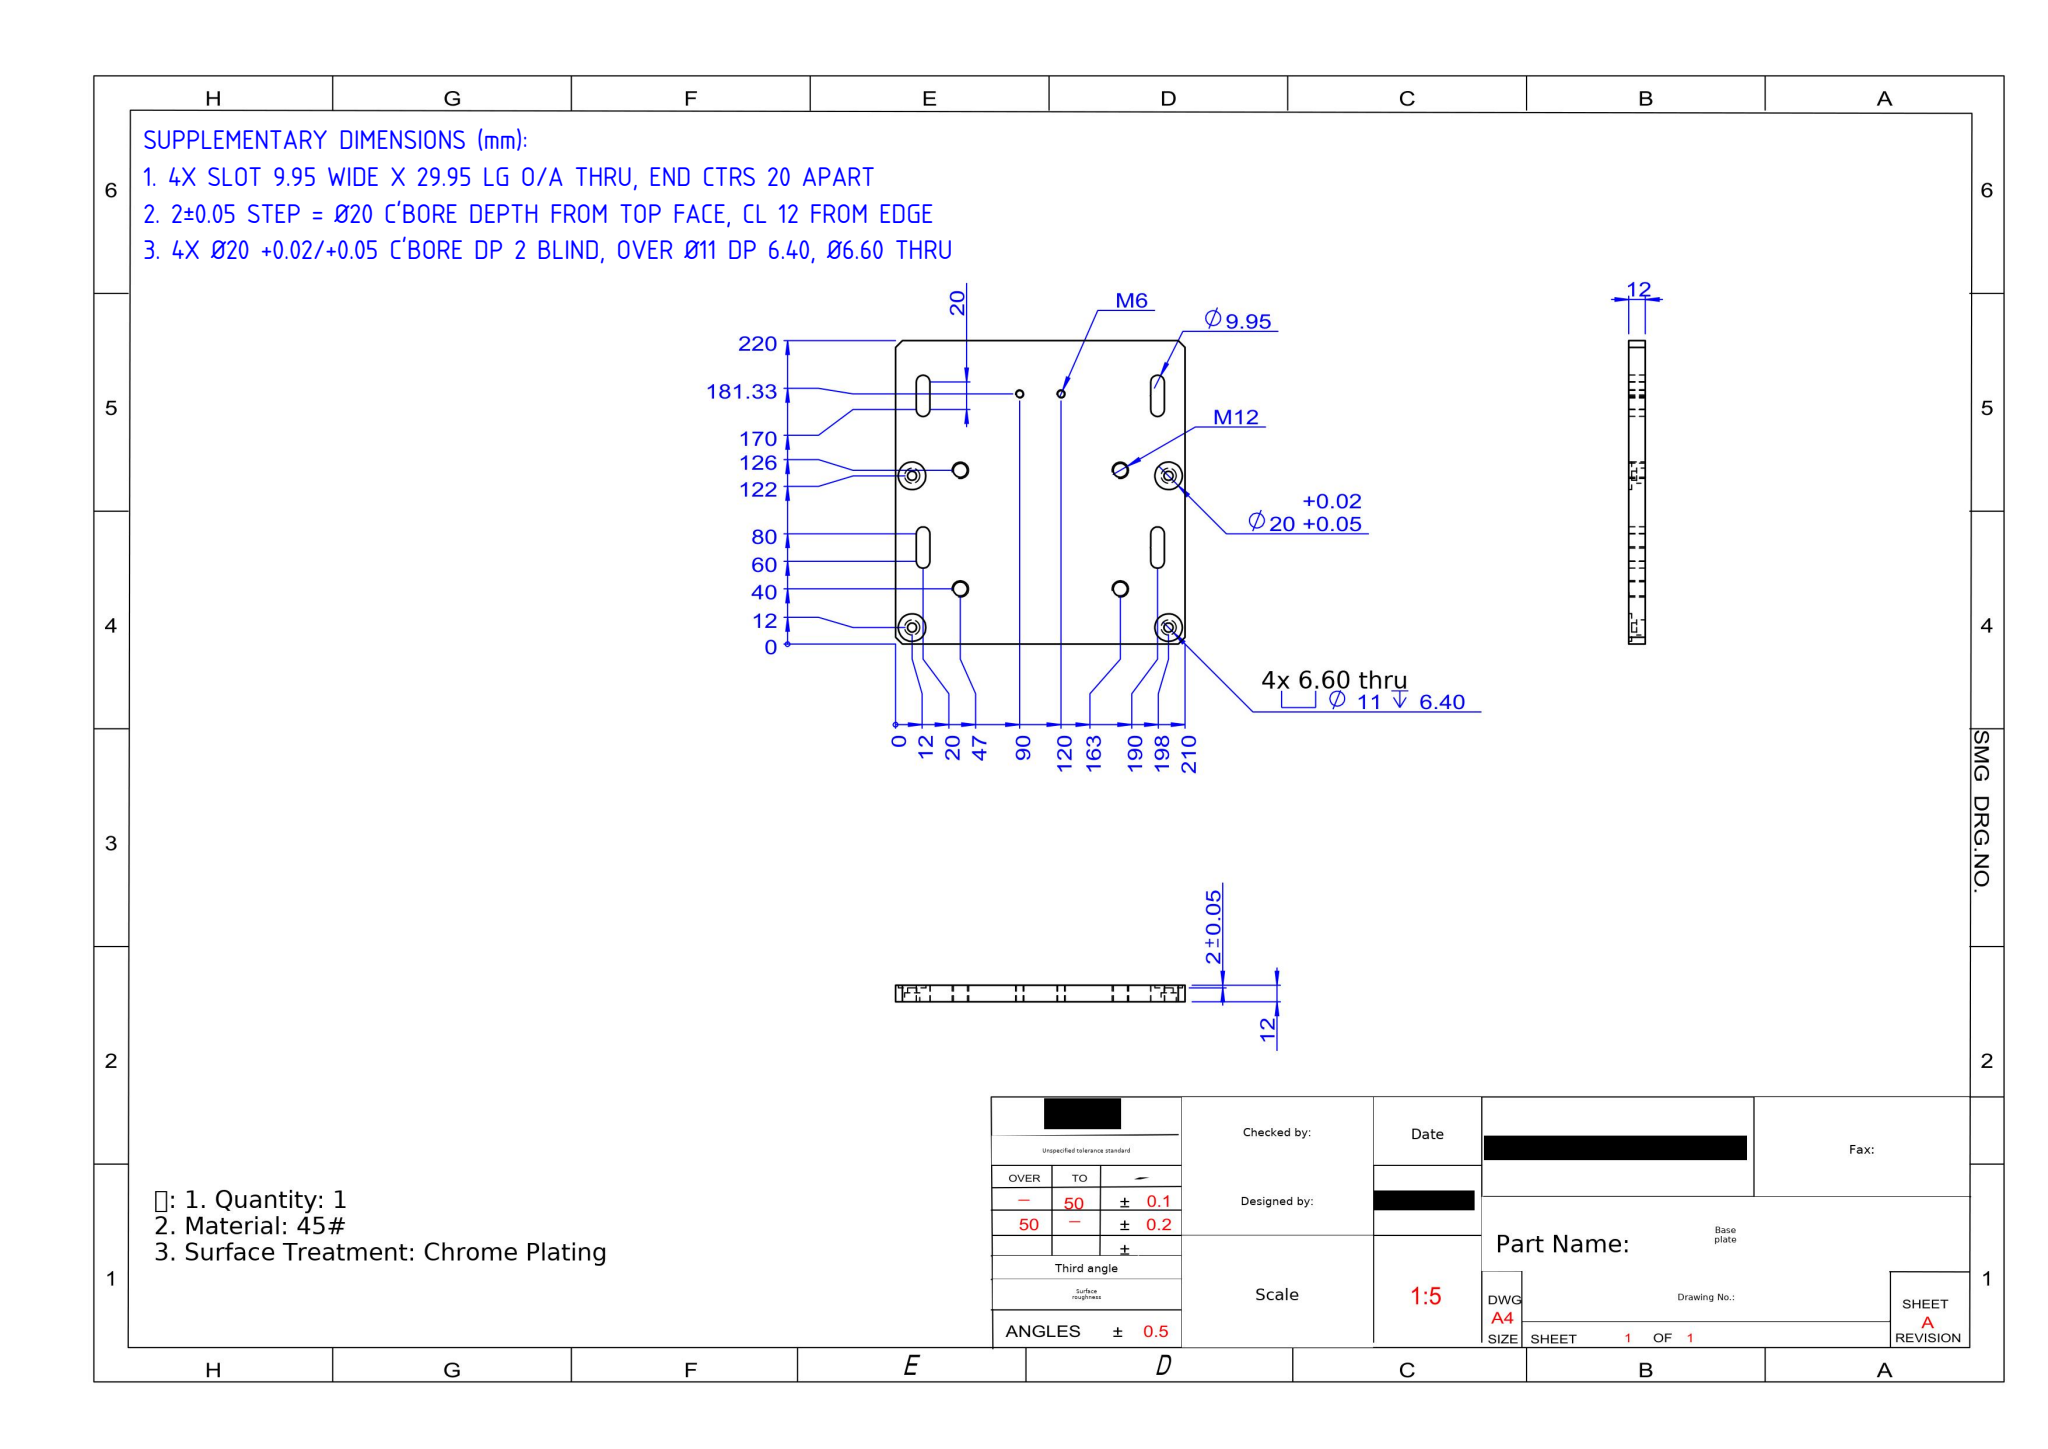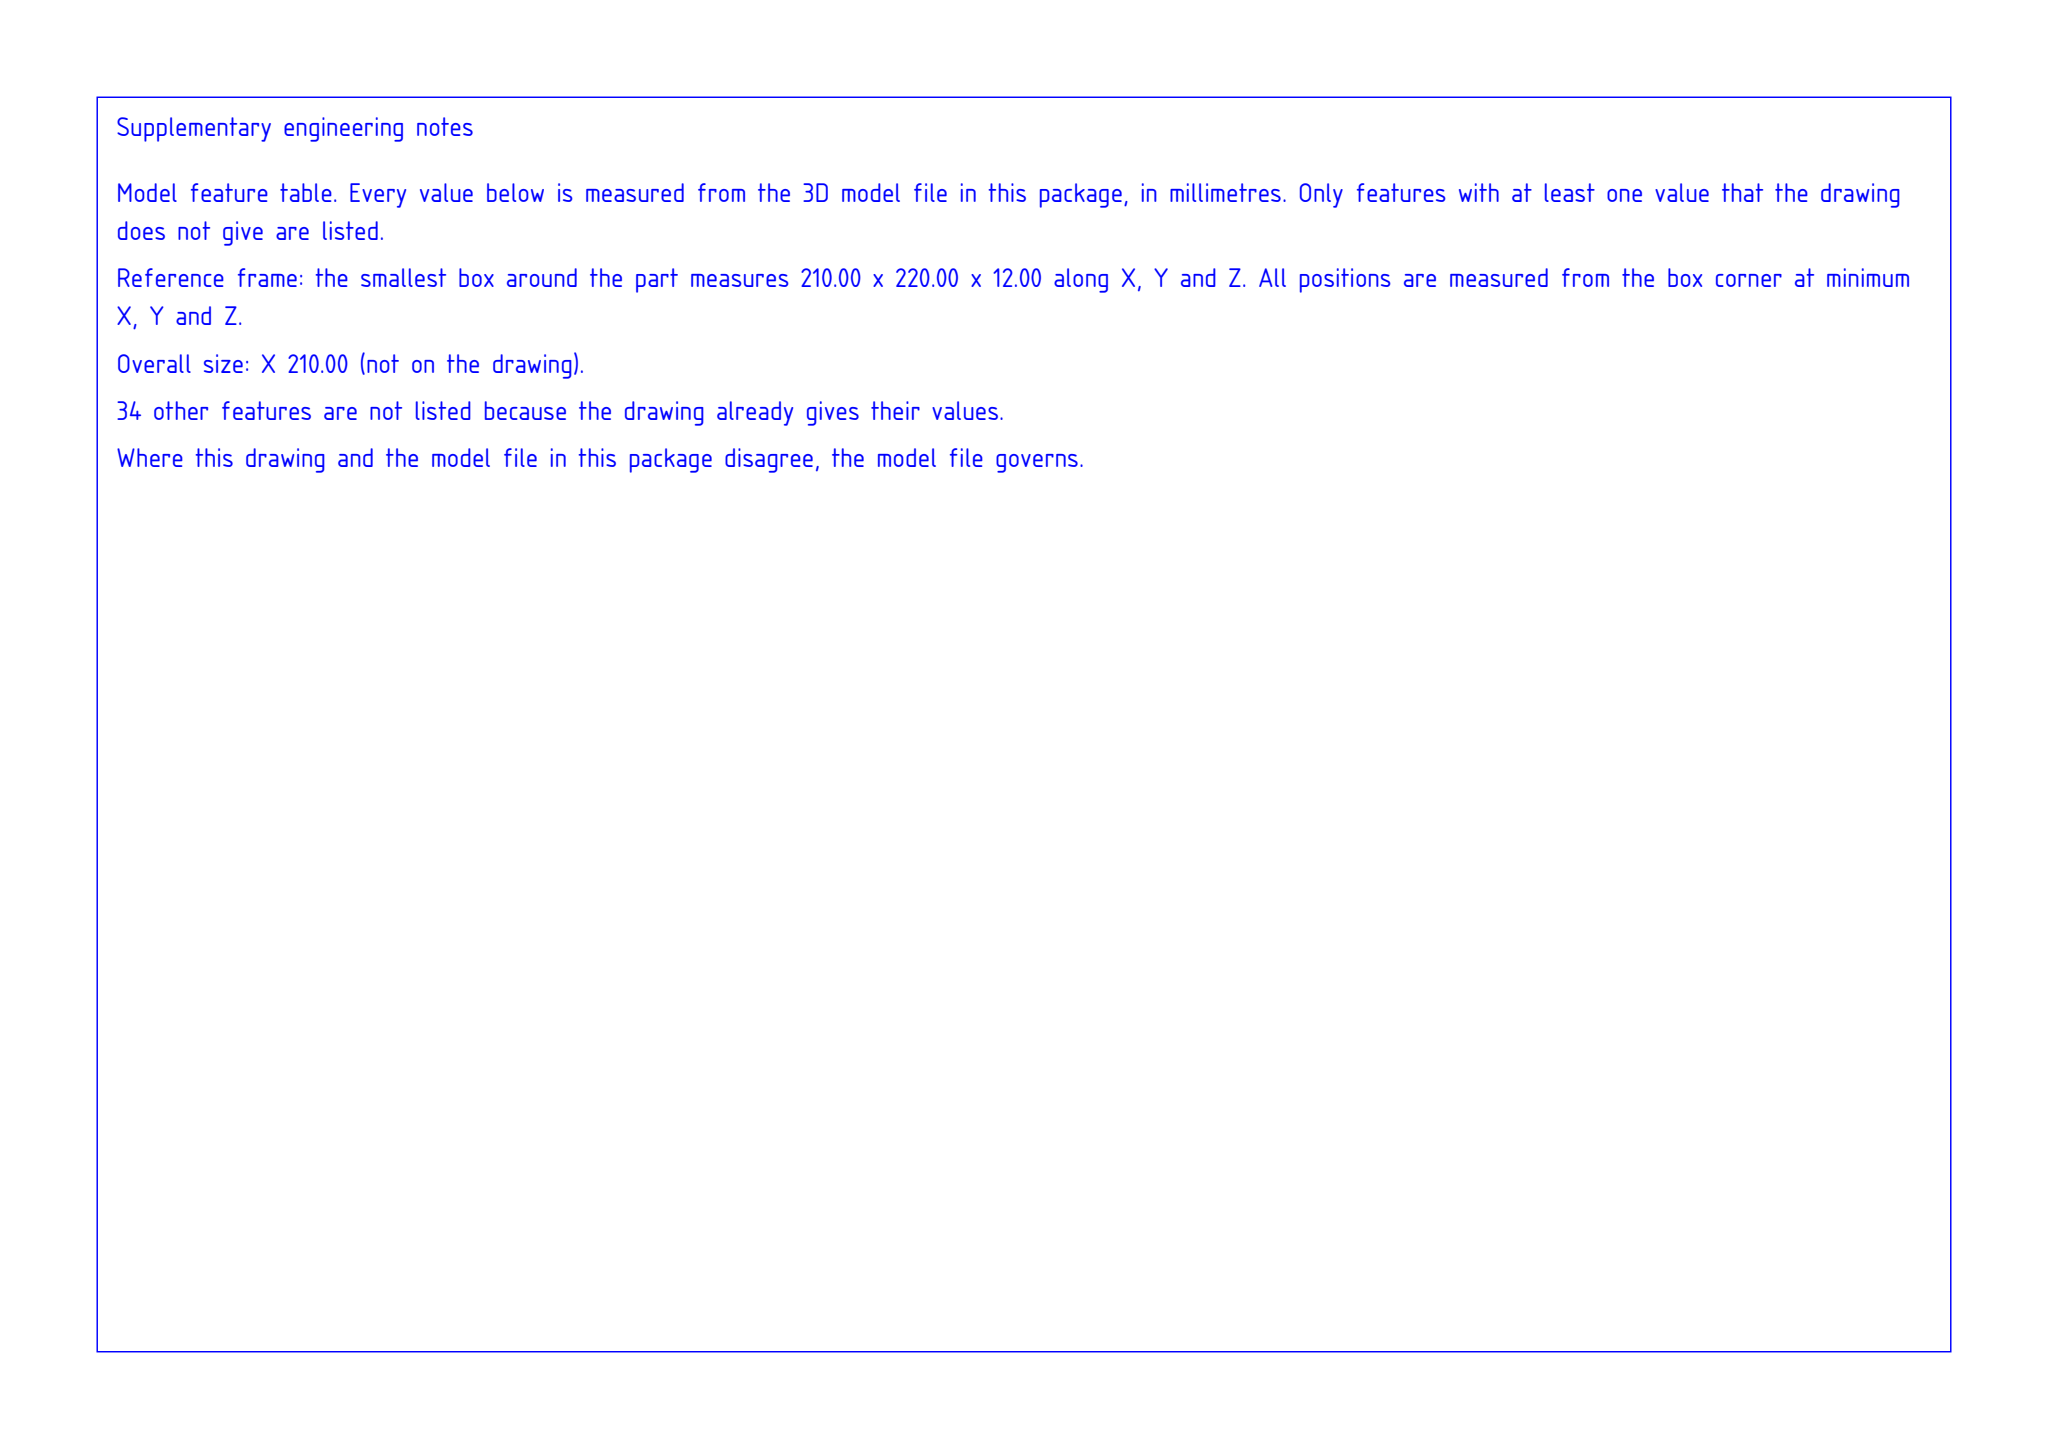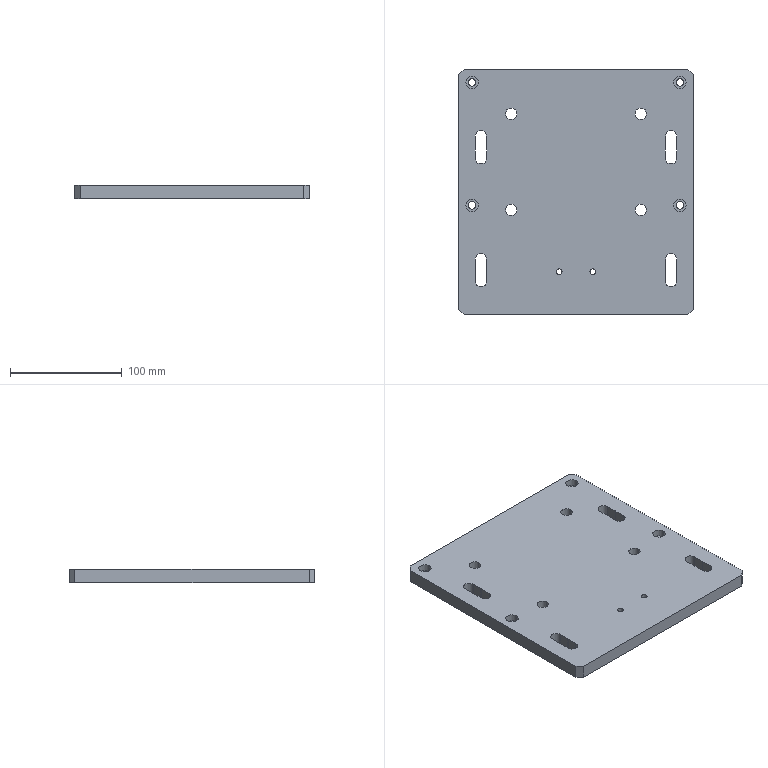Part | SolidWorks | mm | 1 solid | 90 faces | box 210 x 220 x 12 mm | volume 530682 mm3 | cylinder 56 | plane 34 | commonest cylinder face diameters 10 x12 10.2 x8 11 x8 20 x8 6.6 x8 9.95 x8 5 x4